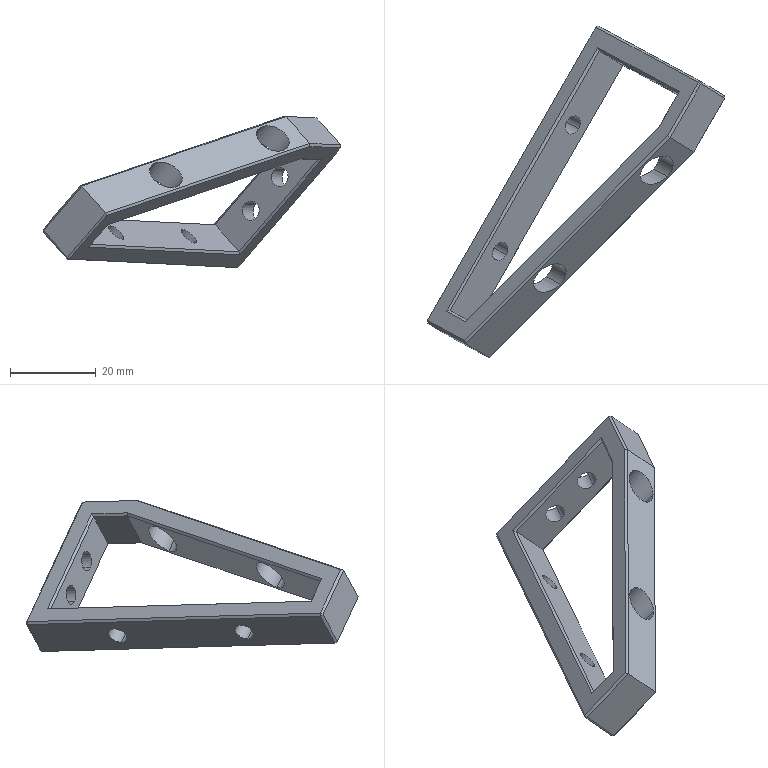Component | SolidWorks | 9z0-123-1 | 1 solid | 53 faces | box 69.41 x 77.52 x 35.27 mm | volume 9054 mm3 | plane 41 | cylinder 12 | commonest cylinder face diameters 4.5 x8 8 x4
build123d program:
from build123d import *

# Parameters (mm, degrees)
BOSS_EXTRUDE1_DEPTH                             = 10
M4_HEX_SOCKET_HEAD_CAP_SCREW_CBORE1_D           = 4.5
M4_HEX_SOCKET_HEAD_CAP_SCREW_CBORE1_CBORE_D     = 8
M4_HEX_SOCKET_HEAD_CAP_SCREW_CBORE1_CBORE_DEPTH = 34.4
SKETCH4_R                                       = 2.25
CUT_EXTRUDE2_DEPTH                              = 10
CHAMFER1_SIZE                                   = 0.5


with BuildPart() as part:
    # Sketch1 → Boss-Extrude1 (new body)
    with BuildSketch(Plane.XY):
        Polygon((-5, 40), (20, -25), (20, -40), (-20, -40), (-20, 40), align=None)
        Polygon((-8.434, 35), (15, -25.928), (15, -35), (-15, -35), (-15, 35), align=None, mode=Mode.SUBTRACT)
    extrude(amount=BOSS_EXTRUDE1_DEPTH)

    # M4 Hex Socket Head Cap Screw CBORE1 (through all)
    with Locations(Plane(origin=(20, 0, 0), x_dir=(0, 0, -1), z_dir=(1, 0, 0))):
        with Locations((-5, -17), (-5, 17)):
            CounterBoreHole(M4_HEX_SOCKET_HEAD_CAP_SCREW_CBORE1_D / 2, M4_HEX_SOCKET_HEAD_CAP_SCREW_CBORE1_CBORE_D / 2, M4_HEX_SOCKET_HEAD_CAP_SCREW_CBORE1_CBORE_DEPTH)

    # Sketch4 → Cut-Extrude2 (cut)
    with BuildSketch(Plane.XZ.offset(40)):
        with Locations(Location((-6, 5, 0), (0, 0, 270))):
            Circle(SKETCH4_R)
        with Locations(Location((5, 5, 0), (0, 0, 270))):
            Circle(SKETCH4_R)
    extrude(amount=-CUT_EXTRUDE2_DEPTH, mode=Mode.SUBTRACT)

    # Chamfer1
    chamfer1_edges = [part.edges().sort_by_distance(p)[0] for p in [
        (-12.5, 40, 10),
        (-20, 0, 10),
        (0, -40, 10),
        (-11.717, 35, 0),
        (-15, 0, 0),
        (0, -35, 0),
        (15, -30.464, 0),
        (3.283, 4.536, 0),
        (-11.717, 35, 10),
        (-15, 0, 10),
        (0, -35, 10),
        (15, -30.464, 10),
        (3.283, 4.536, 10),
        (20, -32.5, 10),
        (0, -40, 0),
        (-20, 0, 0),
        (-12.5, 40, 0),
        (7.5, 7.5, 0),
        (20, -32.5, 0),
        (7.5, 7.5, 10),
        (20, -40, 5),
        (-20, -40, 5),
        (-20, 40, 5),
    ]]
    chamfer(chamfer1_edges, length=CHAMFER1_SIZE)


solid = part.part

# Placed as in the assembly
solid = solid.moved(Location((22.413, -80.921, 172.17), (151.979, 37.728, 38.997)))